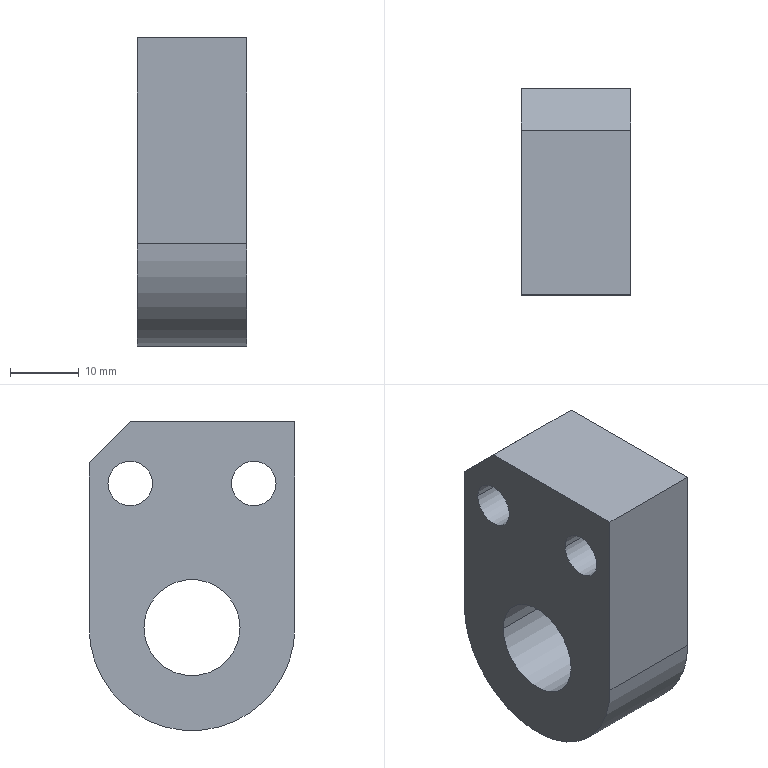Component | SolidWorks | 15LeadScrewPlate-1 | 1 solid | 13 faces | box 16 x 30 x 45 mm | volume 16242 mm3 | cylinder 7 | plane 6 | commonest cylinder face diameters 6.5 x4 14 x2 30 x1
build123d program:
from build123d import *

# Parameters (mm, degrees)
BOSS_EXTRUDE1_DEPTH = 16
SKETCH2_R           = 7
SKETCH2_R_2         = 3.25
CUT_EXTRUDE1_DEPTH  = 80
CUT_EXTRUDE2_DEPTH  = 80


with BuildPart() as part:
    # Sketch1 → Boss-Extrude1 (new body)
    with BuildSketch(Plane.XY):
        with BuildLine():
            Line((15, 0), (15, -30))
            Line((15, -30), (-15, -30))
            Line((-15, -30), (-15, 0))
            ThreePointArc((-15, 0), (0, 15), (15, 0))
        make_face()
    extrude(amount=BOSS_EXTRUDE1_DEPTH)

    # Sketch2 → Cut-Extrude1 (cut)
    with BuildSketch(Plane.XY.offset(16)):
        Circle(SKETCH2_R)
        with Locations((-9, -21)):
            Circle(SKETCH2_R_2)
        with Locations((9, -21)):
            Circle(SKETCH2_R_2)
    extrude(amount=-CUT_EXTRUDE1_DEPTH, mode=Mode.SUBTRACT)

    # Sketch3 → Cut-Extrude2 (cut)
    with BuildSketch(Plane.XY.offset(16)):
        Polygon((-9, -30), (-15, -30), (-15, -24), align=None)
    extrude(amount=-CUT_EXTRUDE2_DEPTH, mode=Mode.SUBTRACT)


solid = part.part

# Placed as in the assembly
solid = solid.moved(Location((-216, 57, -113), (-90, 90, 0)))
STEP:
#1=COLOUR_RGB('',0.7922,0.8196,0.9333);
#2=FILL_AREA_STYLE_COLOUR('',#1);
#3=FILL_AREA_STYLE('',(#2));
#4=SURFACE_STYLE_FILL_AREA(#3);
#5=SURFACE_SIDE_STYLE('',(#4));
#6=SURFACE_STYLE_USAGE(.BOTH.,#5);
#7=PRESENTATION_STYLE_ASSIGNMENT((#6));
#8=CARTESIAN_POINT('',(-8.504,2.52,-4.449));
#9=VERTEX_POINT('',#8);
#10=CARTESIAN_POINT('',(-8.504,1.969,-4.449));
#11=VERTEX_POINT('',#10);
#12=CARTESIAN_POINT('',(-8.504,2.244,-4.449));
#13=DIRECTION('',(1.,0.,-0.));
#14=DIRECTION('',(0.,-1.,-0.));
#15=AXIS2_PLACEMENT_3D('',#12,#13,#14);
#16=CIRCLE('',#15,0.2756);
#17=EDGE_CURVE('',#9,#11,#16,.T.);
#18=ORIENTED_EDGE('',*,*,#17,.F.);
#19=CARTESIAN_POINT('',(-7.874,2.52,-4.449));
#20=VERTEX_POINT('',#19);
#21=CARTESIAN_POINT('',(-11.024,2.52,-4.449));
#22=DIRECTION('',(1.,0.,-0.));
#23=VECTOR('',#22,39.37);
#24=LINE('',#21,#23);
#25=EDGE_CURVE('',#9,#20,#24,.T.);
#26=ORIENTED_EDGE('',*,*,#25,.T.);
#27=CARTESIAN_POINT('',(-7.874,1.969,-4.449));
#28=VERTEX_POINT('',#27);
#29=CARTESIAN_POINT('',(-7.874,2.244,-4.449));
#30=DIRECTION('',(1.,0.,-0.));
#31=DIRECTION('',(0.,-1.,-0.));
#32=AXIS2_PLACEMENT_3D('',#29,#30,#31);
#33=CIRCLE('',#32,0.2756);
#34=EDGE_CURVE('',#20,#28,#33,.T.);
#35=ORIENTED_EDGE('',*,*,#34,.T.);
#36=CARTESIAN_POINT('',(-11.024,1.969,-4.449));
#37=DIRECTION('',(1.,0.,-0.));
#38=VECTOR('',#37,39.37);
#39=LINE('',#36,#38);
#40=EDGE_CURVE('',#11,#28,#39,.T.);
#41=ORIENTED_EDGE('',*,*,#40,.F.);
#42=EDGE_LOOP('',(#18,#26,#35,#41));
#43=FACE_OUTER_BOUND('',#42,.T.);
#44=CARTESIAN_POINT('',(-11.024,2.244,-4.449));
#45=DIRECTION('',(1.,0.,-0.));
#46=DIRECTION('',(0.,-1.,-0.));
#47=AXIS2_PLACEMENT_3D('',#44,#45,#46);
#48=CYLINDRICAL_SURFACE('',#47,0.2756);
#49=ADVANCED_FACE('',(#43),#48,.F.);
#50=CARTESIAN_POINT('',(-8.504,2.726,-3.622));
#51=VERTEX_POINT('',#50);
#52=CARTESIAN_POINT('',(-8.504,2.47,-3.622));
#53=VERTEX_POINT('',#52);
#54=CARTESIAN_POINT('',(-8.504,2.598,-3.622));
#55=DIRECTION('',(1.,0.,-0.));
#56=DIRECTION('',(0.,-1.,-0.));
#57=AXIS2_PLACEMENT_3D('',#54,#55,#56);
#58=CIRCLE('',#57,0.128);
#59=EDGE_CURVE('',#51,#53,#58,.T.);
#60=ORIENTED_EDGE('',*,*,#59,.F.);
#61=CARTESIAN_POINT('',(-7.874,2.726,-3.622));
#62=VERTEX_POINT('',#61);
#63=CARTESIAN_POINT('',(-11.024,2.726,-3.622));
#64=DIRECTION('',(1.,0.,-0.));
#65=VECTOR('',#64,39.37);
#66=LINE('',#63,#65);
#67=EDGE_CURVE('',#51,#62,#66,.T.);
#68=ORIENTED_EDGE('',*,*,#67,.T.);
#69=CARTESIAN_POINT('',(-7.874,2.47,-3.622));
#70=VERTEX_POINT('',#69);
#71=CARTESIAN_POINT('',(-7.874,2.598,-3.622));
#72=DIRECTION('',(1.,0.,-0.));
#73=DIRECTION('',(0.,-1.,-0.));
#74=AXIS2_PLACEMENT_3D('',#71,#72,#73);
#75=CIRCLE('',#74,0.128);
#76=EDGE_CURVE('',#62,#70,#75,.T.);
#77=ORIENTED_EDGE('',*,*,#76,.T.);
#78=CARTESIAN_POINT('',(-11.024,2.47,-3.622));
#79=DIRECTION('',(1.,0.,-0.));
#80=VECTOR('',#79,39.37);
#81=LINE('',#78,#80);
#82=EDGE_CURVE('',#53,#70,#81,.T.);
#83=ORIENTED_EDGE('',*,*,#82,.F.);
#84=EDGE_LOOP('',(#60,#68,#77,#83));
#85=FACE_OUTER_BOUND('',#84,.T.);
#86=CARTESIAN_POINT('',(-11.024,2.598,-3.622));
#87=DIRECTION('',(1.,0.,-0.));
#88=DIRECTION('',(0.,-1.,-0.));
#89=AXIS2_PLACEMENT_3D('',#86,#87,#88);
#90=CYLINDRICAL_SURFACE('',#89,0.128);
#91=ADVANCED_FACE('',(#85),#90,.F.);
#92=CARTESIAN_POINT('',(-8.504,2.018,-3.622));
#93=VERTEX_POINT('',#92);
#94=CARTESIAN_POINT('',(-8.504,1.762,-3.622));
#95=VERTEX_POINT('',#94);
#96=CARTESIAN_POINT('',(-8.504,1.89,-3.622));
#97=DIRECTION('',(1.,0.,-0.));
#98=DIRECTION('',(0.,-1.,-0.));
#99=AXIS2_PLACEMENT_3D('',#96,#97,#98);
#100=CIRCLE('',#99,0.128);
#101=EDGE_CURVE('',#93,#95,#100,.T.);
#102=ORIENTED_EDGE('',*,*,#101,.F.);
#103=CARTESIAN_POINT('',(-7.874,2.018,-3.622));
#104=VERTEX_POINT('',#103);
#105=CARTESIAN_POINT('',(-11.024,2.018,-3.622));
#106=DIRECTION('',(1.,0.,-0.));
#107=VECTOR('',#106,39.37);
#108=LINE('',#105,#107);
#109=EDGE_CURVE('',#93,#104,#108,.T.);
#110=ORIENTED_EDGE('',*,*,#109,.T.);
#111=CARTESIAN_POINT('',(-7.874,1.762,-3.622));
#112=VERTEX_POINT('',#111);
#113=CARTESIAN_POINT('',(-7.874,1.89,-3.622));
#114=DIRECTION('',(1.,0.,-0.));
#115=DIRECTION('',(0.,1.,0.));
#116=AXIS2_PLACEMENT_3D('',#113,#114,#115);
#117=CIRCLE('',#116,0.128);
#118=EDGE_CURVE('',#104,#112,#117,.T.);
#119=ORIENTED_EDGE('',*,*,#118,.T.);
#120=CARTESIAN_POINT('',(-11.024,1.762,-3.622));
#121=DIRECTION('',(1.,0.,-0.));
#122=VECTOR('',#121,39.37);
#123=LINE('',#120,#122);
#124=EDGE_CURVE('',#95,#112,#123,.T.);
#125=ORIENTED_EDGE('',*,*,#124,.F.);
#126=EDGE_LOOP('',(#102,#110,#119,#125));
#127=FACE_OUTER_BOUND('',#126,.T.);
#128=CARTESIAN_POINT('',(-11.024,1.89,-3.622));
#129=DIRECTION('',(1.,0.,-0.));
#130=DIRECTION('',(0.,-1.,-0.));
#131=AXIS2_PLACEMENT_3D('',#128,#129,#130);
#132=CYLINDRICAL_SURFACE('',#131,0.128);
#133=ADVANCED_FACE('',(#127),#132,.F.);
#134=CARTESIAN_POINT('',(-7.874,2.598,-3.268));
#135=VERTEX_POINT('',#134);
#136=CARTESIAN_POINT('',(-7.874,1.654,-3.268));
#137=VERTEX_POINT('',#136);
#138=CARTESIAN_POINT('',(-7.874,2.244,-3.268));
#139=DIRECTION('',(0.,-1.,-0.));
#140=VECTOR('',#139,39.37);
#141=LINE('',#138,#140);
#142=EDGE_CURVE('',#135,#137,#141,.T.);
#143=ORIENTED_EDGE('',*,*,#142,.F.);
#144=CARTESIAN_POINT('',(-8.504,2.598,-3.268));
#145=VERTEX_POINT('',#144);
#146=CARTESIAN_POINT('',(-11.024,2.598,-3.268));
#147=DIRECTION('',(1.,0.,-0.));
#148=VECTOR('',#147,39.37);
#149=LINE('',#146,#148);
#150=EDGE_CURVE('',#145,#135,#149,.T.);
#151=ORIENTED_EDGE('',*,*,#150,.F.);
#152=CARTESIAN_POINT('',(-8.504,1.654,-3.268));
#153=VERTEX_POINT('',#152);
#154=CARTESIAN_POINT('',(-8.504,2.244,-3.268));
#155=DIRECTION('',(0.,-1.,-0.));
#156=VECTOR('',#155,39.37);
#157=LINE('',#154,#156);
#158=EDGE_CURVE('',#145,#153,#157,.T.);
#159=ORIENTED_EDGE('',*,*,#158,.T.);
#160=CARTESIAN_POINT('',(-7.874,1.654,-3.268));
#161=DIRECTION('',(-1.,-0.,0.));
#162=VECTOR('',#161,39.37);
#163=LINE('',#160,#162);
#164=EDGE_CURVE('',#137,#153,#163,.T.);
#165=ORIENTED_EDGE('',*,*,#164,.F.);
#166=EDGE_LOOP('',(#143,#151,#159,#165));
#167=FACE_OUTER_BOUND('',#166,.T.);
#168=CARTESIAN_POINT('',(-7.874,2.244,-3.268));
#169=DIRECTION('',(-0.,0.,-1.));
#170=DIRECTION('',(-0.,1.,0.));
#171=AXIS2_PLACEMENT_3D('',#168,#169,#170);
#172=PLANE('',#171);
#173=ADVANCED_FACE('',(#167),#172,.F.);
#174=CARTESIAN_POINT('',(-8.504,1.654,-4.449));
#175=VERTEX_POINT('',#174);
#176=CARTESIAN_POINT('',(-8.504,1.654,-4.449));
#177=DIRECTION('',(0.,-0.,1.));
#178=VECTOR('',#177,39.37);
#179=LINE('',#176,#178);
#180=EDGE_CURVE('',#175,#153,#179,.T.);
#181=ORIENTED_EDGE('',*,*,#180,.F.);
#182=CARTESIAN_POINT('',(-7.874,1.654,-4.449));
#183=VERTEX_POINT('',#182);
#184=CARTESIAN_POINT('',(-7.874,1.654,-4.449));
#185=DIRECTION('',(-1.,-0.,0.));
#186=VECTOR('',#185,39.37);
#187=LINE('',#184,#186);
#188=EDGE_CURVE('',#183,#175,#187,.T.);
#189=ORIENTED_EDGE('',*,*,#188,.F.);
#190=CARTESIAN_POINT('',(-7.874,1.654,-4.449));
#191=DIRECTION('',(0.,-0.,1.));
#192=VECTOR('',#191,39.37);
#193=LINE('',#190,#192);
#194=EDGE_CURVE('',#183,#137,#193,.T.);
#195=ORIENTED_EDGE('',*,*,#194,.T.);
#196=ORIENTED_EDGE('',*,*,#164,.T.);
#197=EDGE_LOOP('',(#181,#189,#195,#196));
#198=FACE_OUTER_BOUND('',#197,.T.);
#199=CARTESIAN_POINT('',(-7.874,1.654,-4.449));
#200=DIRECTION('',(0.,-1.,-0.));
#201=DIRECTION('',(-0.,0.,-1.));
#202=AXIS2_PLACEMENT_3D('',#199,#200,#201);
#203=PLANE('',#202);
#204=ADVANCED_FACE('',(#198),#203,.T.);
#205=CARTESIAN_POINT('',(-8.504,2.835,-4.449));
#206=VERTEX_POINT('',#205);
#207=CARTESIAN_POINT('',(-8.504,2.244,-4.449));
#208=DIRECTION('',(1.,0.,-0.));
#209=DIRECTION('',(0.,-1.,-0.));
#210=AXIS2_PLACEMENT_3D('',#207,#208,#209);
#211=CIRCLE('',#210,0.5906);
#212=EDGE_CURVE('',#175,#206,#211,.T.);
#213=ORIENTED_EDGE('',*,*,#212,.T.);
#214=CARTESIAN_POINT('',(-7.874,2.835,-4.449));
#215=VERTEX_POINT('',#214);
#216=CARTESIAN_POINT('',(-7.874,2.835,-4.449));
#217=DIRECTION('',(-1.,-0.,0.));
#218=VECTOR('',#217,39.37);
#219=LINE('',#216,#218);
#220=EDGE_CURVE('',#215,#206,#219,.T.);
#221=ORIENTED_EDGE('',*,*,#220,.F.);
#222=CARTESIAN_POINT('',(-7.874,2.244,-4.449));
#223=DIRECTION('',(1.,0.,-0.));
#224=DIRECTION('',(0.,-1.,-0.));
#225=AXIS2_PLACEMENT_3D('',#222,#223,#224);
#226=CIRCLE('',#225,0.5906);
#227=EDGE_CURVE('',#183,#215,#226,.T.);
#228=ORIENTED_EDGE('',*,*,#227,.F.);
#229=ORIENTED_EDGE('',*,*,#188,.T.);
#230=EDGE_LOOP('',(#213,#221,#228,#229));
#231=FACE_OUTER_BOUND('',#230,.T.);
#232=CARTESIAN_POINT('',(-7.874,2.244,-4.449));
#233=DIRECTION('',(-1.,-0.,0.));
#234=DIRECTION('',(-0.,1.,0.));
#235=AXIS2_PLACEMENT_3D('',#232,#233,#234);
#236=CYLINDRICAL_SURFACE('',#235,0.5906);
#237=ADVANCED_FACE('',(#231),#236,.T.);
#238=CARTESIAN_POINT('',(-8.504,2.835,-3.504));
#239=VERTEX_POINT('',#238);
#240=CARTESIAN_POINT('',(-8.504,2.835,-4.449));
#241=DIRECTION('',(0.,-0.,1.));
#242=VECTOR('',#241,39.37);
#243=LINE('',#240,#242);
#244=EDGE_CURVE('',#206,#239,#243,.T.);
#245=ORIENTED_EDGE('',*,*,#244,.T.);
#246=CARTESIAN_POINT('',(-7.874,2.835,-3.504));
#247=VERTEX_POINT('',#246);
#248=CARTESIAN_POINT('',(-11.024,2.835,-3.504));
#249=DIRECTION('',(1.,0.,-0.));
#250=VECTOR('',#249,39.37);
#251=LINE('',#248,#250);
#252=EDGE_CURVE('',#239,#247,#251,.T.);
#253=ORIENTED_EDGE('',*,*,#252,.T.);
#254=CARTESIAN_POINT('',(-7.874,2.835,-4.449));
#255=DIRECTION('',(0.,-0.,1.));
#256=VECTOR('',#255,39.37);
#257=LINE('',#254,#256);
#258=EDGE_CURVE('',#215,#247,#257,.T.);
#259=ORIENTED_EDGE('',*,*,#258,.F.);
#260=ORIENTED_EDGE('',*,*,#220,.T.);
#261=EDGE_LOOP('',(#245,#253,#259,#260));
#262=FACE_OUTER_BOUND('',#261,.T.);
#263=CARTESIAN_POINT('',(-7.874,2.835,-4.449));
#264=DIRECTION('',(0.,-1.,-0.));
#265=DIRECTION('',(-0.,0.,-1.));
#266=AXIS2_PLACEMENT_3D('',#263,#264,#265);
#267=PLANE('',#266);
#268=ADVANCED_FACE('',(#262),#267,.F.);
#269=CARTESIAN_POINT('',(-7.874,2.835,-3.504));
#270=DIRECTION('',(-0.,0.7071,-0.7071));
#271=VECTOR('',#270,39.37);
#272=LINE('',#269,#271);
#273=EDGE_CURVE('',#135,#247,#272,.T.);
#274=ORIENTED_EDGE('',*,*,#273,.F.);
#275=ORIENTED_EDGE('',*,*,#142,.T.);
#276=ORIENTED_EDGE('',*,*,#194,.F.);
#277=ORIENTED_EDGE('',*,*,#227,.T.);
#278=ORIENTED_EDGE('',*,*,#258,.T.);
#279=EDGE_LOOP('',(#274,#275,#276,#277,#278));
#280=FACE_OUTER_BOUND('',#279,.T.);
#281=CARTESIAN_POINT('',(-7.874,2.244,-4.449));
#282=DIRECTION('',(1.,0.,-0.));
#283=DIRECTION('',(0.,-1.,-0.));
#284=AXIS2_PLACEMENT_3D('',#281,#282,#283);
#285=CIRCLE('',#284,0.2756);
#286=EDGE_CURVE('',#28,#20,#285,.T.);
#287=ORIENTED_EDGE('',*,*,#286,.F.);
#288=ORIENTED_EDGE('',*,*,#34,.F.);
#289=EDGE_LOOP('',(#287,#288));
#290=FACE_BOUND('',#289,.T.);
#291=CARTESIAN_POINT('',(-7.874,2.598,-3.622));
#292=DIRECTION('',(1.,0.,-0.));
#293=DIRECTION('',(0.,-1.,-0.));
#294=AXIS2_PLACEMENT_3D('',#291,#292,#293);
#295=CIRCLE('',#294,0.128);
#296=EDGE_CURVE('',#70,#62,#295,.T.);
#297=ORIENTED_EDGE('',*,*,#296,.F.);
#298=ORIENTED_EDGE('',*,*,#76,.F.);
#299=EDGE_LOOP('',(#297,#298));
#300=FACE_BOUND('',#299,.T.);
#301=CARTESIAN_POINT('',(-7.874,1.89,-3.622));
#302=DIRECTION('',(1.,0.,-0.));
#303=DIRECTION('',(0.,1.,0.));
#304=AXIS2_PLACEMENT_3D('',#301,#302,#303);
#305=CIRCLE('',#304,0.128);
#306=EDGE_CURVE('',#112,#104,#305,.T.);
#307=ORIENTED_EDGE('',*,*,#306,.F.);
#308=ORIENTED_EDGE('',*,*,#118,.F.);
#309=EDGE_LOOP('',(#307,#308));
#310=FACE_BOUND('',#309,.T.);
#311=CARTESIAN_POINT('',(-7.874,2.244,-4.449));
#312=DIRECTION('',(1.,0.,-0.));
#313=DIRECTION('',(0.,-1.,-0.));
#314=AXIS2_PLACEMENT_3D('',#311,#312,#313);
#315=PLANE('',#314);
#316=ADVANCED_FACE('',(#280,#290,#300,#310),#315,.T.);
#317=CARTESIAN_POINT('',(-8.504,2.244,-4.449));
#318=DIRECTION('',(1.,0.,-0.));
#319=DIRECTION('',(0.,-1.,-0.));
#320=AXIS2_PLACEMENT_3D('',#317,#318,#319);
#321=CIRCLE('',#320,0.2756);
#322=EDGE_CURVE('',#11,#9,#321,.T.);
#323=ORIENTED_EDGE('',*,*,#322,.T.);
#324=ORIENTED_EDGE('',*,*,#17,.T.);
#325=EDGE_LOOP('',(#323,#324));
#326=FACE_BOUND('',#325,.T.);
#327=CARTESIAN_POINT('',(-8.504,2.598,-3.622));
#328=DIRECTION('',(1.,0.,-0.));
#329=DIRECTION('',(0.,-1.,-0.));
#330=AXIS2_PLACEMENT_3D('',#327,#328,#329);
#331=CIRCLE('',#330,0.128);
#332=EDGE_CURVE('',#53,#51,#331,.T.);
#333=ORIENTED_EDGE('',*,*,#332,.T.);
#334=ORIENTED_EDGE('',*,*,#59,.T.);
#335=EDGE_LOOP('',(#333,#334));
#336=FACE_BOUND('',#335,.T.);
#337=CARTESIAN_POINT('',(-8.504,1.89,-3.622));
#338=DIRECTION('',(1.,0.,-0.));
#339=DIRECTION('',(0.,-1.,-0.));
#340=AXIS2_PLACEMENT_3D('',#337,#338,#339);
#341=CIRCLE('',#340,0.128);
#342=EDGE_CURVE('',#95,#93,#341,.T.);
#343=ORIENTED_EDGE('',*,*,#342,.T.);
#344=ORIENTED_EDGE('',*,*,#101,.T.);
#345=EDGE_LOOP('',(#343,#344));
#346=FACE_BOUND('',#345,.T.);
#347=ORIENTED_EDGE('',*,*,#158,.F.);
#348=CARTESIAN_POINT('',(-8.504,3.012,-3.681));
#349=DIRECTION('',(-0.,0.7071,-0.7071));
#350=VECTOR('',#349,39.37);
#351=LINE('',#348,#350);
#352=EDGE_CURVE('',#145,#239,#351,.T.);
#353=ORIENTED_EDGE('',*,*,#352,.T.);
#354=ORIENTED_EDGE('',*,*,#244,.F.);
#355=ORIENTED_EDGE('',*,*,#212,.F.);
#356=ORIENTED_EDGE('',*,*,#180,.T.);
#357=EDGE_LOOP('',(#347,#353,#354,#355,#356));
#358=FACE_OUTER_BOUND('',#357,.T.);
#359=CARTESIAN_POINT('',(-8.504,2.244,-4.449));
#360=DIRECTION('',(1.,0.,-0.));
#361=DIRECTION('',(0.,-1.,-0.));
#362=AXIS2_PLACEMENT_3D('',#359,#360,#361);
#363=PLANE('',#362);
#364=ADVANCED_FACE('',(#326,#336,#346,#358),#363,.F.);
#365=ORIENTED_EDGE('',*,*,#109,.F.);
#366=ORIENTED_EDGE('',*,*,#342,.F.);
#367=ORIENTED_EDGE('',*,*,#124,.T.);
#368=ORIENTED_EDGE('',*,*,#306,.T.);
#369=EDGE_LOOP('',(#365,#366,#367,#368));
#370=FACE_OUTER_BOUND('',#369,.T.);
#371=CARTESIAN_POINT('',(-11.024,1.89,-3.622));
#372=DIRECTION('',(1.,0.,-0.));
#373=DIRECTION('',(0.,-1.,-0.));
#374=AXIS2_PLACEMENT_3D('',#371,#372,#373);
#375=CYLINDRICAL_SURFACE('',#374,0.128);
#376=ADVANCED_FACE('',(#370),#375,.F.);
#377=ORIENTED_EDGE('',*,*,#67,.F.);
#378=ORIENTED_EDGE('',*,*,#332,.F.);
#379=ORIENTED_EDGE('',*,*,#82,.T.);
#380=ORIENTED_EDGE('',*,*,#296,.T.);
#381=EDGE_LOOP('',(#377,#378,#379,#380));
#382=FACE_OUTER_BOUND('',#381,.T.);
#383=CARTESIAN_POINT('',(-11.024,2.598,-3.622));
#384=DIRECTION('',(1.,0.,-0.));
#385=DIRECTION('',(0.,-1.,-0.));
#386=AXIS2_PLACEMENT_3D('',#383,#384,#385);
#387=CYLINDRICAL_SURFACE('',#386,0.128);
#388=ADVANCED_FACE('',(#382),#387,.F.);
#389=ORIENTED_EDGE('',*,*,#25,.F.);
#390=ORIENTED_EDGE('',*,*,#322,.F.);
#391=ORIENTED_EDGE('',*,*,#40,.T.);
#392=ORIENTED_EDGE('',*,*,#286,.T.);
#393=EDGE_LOOP('',(#389,#390,#391,#392));
#394=FACE_OUTER_BOUND('',#393,.T.);
#395=CARTESIAN_POINT('',(-11.024,2.244,-4.449));
#396=DIRECTION('',(1.,0.,-0.));
#397=DIRECTION('',(0.,-1.,-0.));
#398=AXIS2_PLACEMENT_3D('',#395,#396,#397);
#399=CYLINDRICAL_SURFACE('',#398,0.2756);
#400=ADVANCED_FACE('',(#394),#399,.F.);
#401=ORIENTED_EDGE('',*,*,#150,.T.);
#402=ORIENTED_EDGE('',*,*,#273,.T.);
#403=ORIENTED_EDGE('',*,*,#252,.F.);
#404=ORIENTED_EDGE('',*,*,#352,.F.);
#405=EDGE_LOOP('',(#401,#402,#403,#404));
#406=FACE_OUTER_BOUND('',#405,.T.);
#407=CARTESIAN_POINT('',(-11.024,2.835,-3.504));
#408=DIRECTION('',(-0.,-0.7071,-0.7071));
#409=DIRECTION('',(-0.,0.7071,-0.7071));
#410=AXIS2_PLACEMENT_3D('',#407,#408,#409);
#411=PLANE('',#410);
#412=ADVANCED_FACE('',(#406),#411,.F.);
#413=CLOSED_SHELL('',(#49,#91,#133,#173,#204,#237,#268,#316,#364,#376,#388,#400,#412));
#414=MANIFOLD_SOLID_BREP('',#413);
#415=STYLED_ITEM('',(#7),#414);
#416=(LENGTH_UNIT()NAMED_UNIT(*)SI_UNIT($,.METRE.));
#417=LENGTH_MEASURE_WITH_UNIT(LENGTH_MEASURE(0.0254),#416);
#418=DIMENSIONAL_EXPONENTS(1.,0.,0.,0.,0.,0.,0.);
#419=(CONVERSION_BASED_UNIT('',#417)LENGTH_UNIT()NAMED_UNIT(#418));
#420=UNCERTAINTY_MEASURE_WITH_UNIT(LENGTH_MEASURE(0.00001),#419,'','');
#421=(NAMED_UNIT(*)PLANE_ANGLE_UNIT()SI_UNIT($,.RADIAN.));
#422=(NAMED_UNIT(*)SI_UNIT($,.STERADIAN.)SOLID_ANGLE_UNIT());
#423=(GEOMETRIC_REPRESENTATION_CONTEXT(3)GLOBAL_UNCERTAINTY_ASSIGNED_CONTEXT((#420))GLOBAL_UNIT_ASSIGNED_CONTEXT((#419,#421,#422))REPRESENTATION_CONTEXT('',''));
#424=MECHANICAL_DESIGN_GEOMETRIC_PRESENTATION_REPRESENTATION('',(#415),#423);
#425=CARTESIAN_POINT('',(0.,0.,0.));
#426=DIRECTION('',(0.,0.,1.));
#427=DIRECTION('',(1.,0.,0.));
#428=AXIS2_PLACEMENT_3D('',#425,#426,#427);
#429=(LENGTH_UNIT()NAMED_UNIT(*)SI_UNIT($,.METRE.));
#430=LENGTH_MEASURE_WITH_UNIT(LENGTH_MEASURE(0.0254),#429);
#431=DIMENSIONAL_EXPONENTS(1.,0.,0.,0.,0.,0.,0.);
#432=(CONVERSION_BASED_UNIT('',#430)LENGTH_UNIT()NAMED_UNIT(#431));
#433=UNCERTAINTY_MEASURE_WITH_UNIT(LENGTH_MEASURE(0.00001),#432,'','');
#434=(NAMED_UNIT(*)PLANE_ANGLE_UNIT()SI_UNIT($,.RADIAN.));
#435=(NAMED_UNIT(*)SI_UNIT($,.STERADIAN.)SOLID_ANGLE_UNIT());
#436=(GEOMETRIC_REPRESENTATION_CONTEXT(3)GLOBAL_UNCERTAINTY_ASSIGNED_CONTEXT((#433))GLOBAL_UNIT_ASSIGNED_CONTEXT((#432,#434,#435))REPRESENTATION_CONTEXT('',''));
#437=ADVANCED_BREP_SHAPE_REPRESENTATION('',(#414,#428),#436);
#438=PRESENTATION_LAYER_ASSIGNMENT('','',(#415));